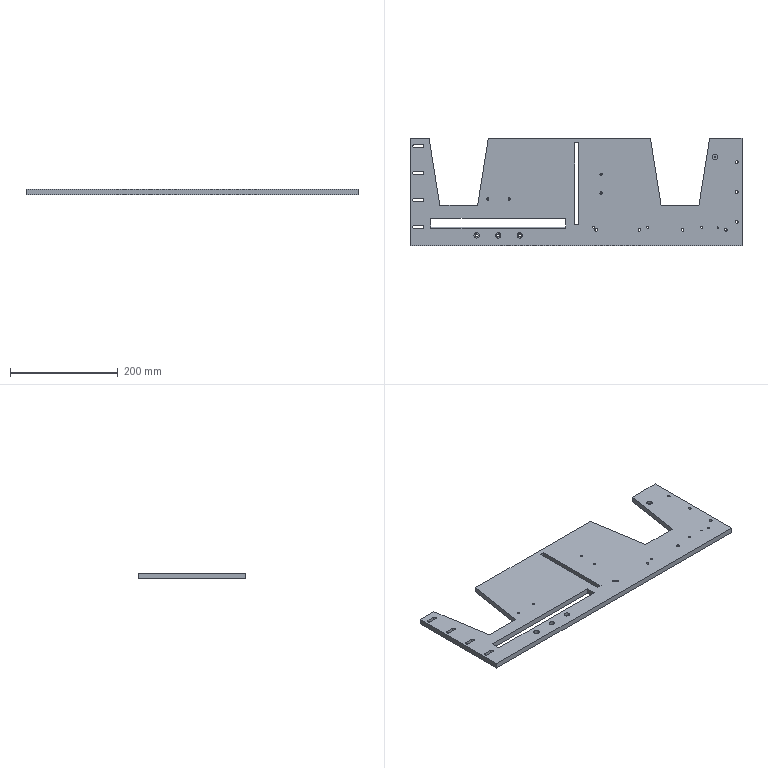Component | SolidWorks | P-SLJ-001-009-2 | 1 solid | 93 faces | box 615 x 200 x 10 mm | volume 943482 mm3 | cylinder 58 | plane 35 | commonest cylinder face diameters 5.5 x24 3.3 x8 10 x8 4.2 x8 5 x8 2.5 x2 | material A3
build123d program:
from build123d import *

# Parameters (mm, degrees)
SKETCH1_W                                            = 615
SKETCH1_H                                            = 200
EXTRUDE1_DEPTH                                       = 5
TAP_DRILL_FOR_M4X0_5_TAP1_D                          = 5.5
EXTRUDE2_DEPTH                                       = 324.506
M6_TAPPED_HOLE1_D                                    = 5
SKETCH9_W                                            = 8
SKETCH9_H                                            = 151
EXTRUDE3_DEPTH                                       = 324.506
EXTRUDE4_DEPTH                                       = 324.506
M5_TAPPED_HOLE1_2_D                                  = 4.2
HOLE_SIZE_ACCORDING_TO_TYPE_OF_HEX_SOCKE_D           = 5.5
HOLE_SIZE_ACCORDING_TO_TYPE_OF_HEX_SOCKE_CBORE_D     = 10
HOLE_SIZE_ACCORDING_TO_TYPE_OF_HEX_SOCKE_CBORE_DEPTH = 5.7
SKETCH16_W                                           = 250
SKETCH16_H                                           = 16
EXTRUDE5_DEPTH                                       = 324.506
M5_TAPPED_HOLE1_D                                    = 4.2
CHAMFER1_SIZE                                        = 2
CHAMFER1_SIZE2                                       = 5
M4_TAPPED_HOLE3_D                                    = 3.3
SKETCH25_R                                           = 5
EXTRUDE6_DEPTH                                       = 5
M4_TAPPED_HOLE4_D                                    = 3.3
M3_TAPPED_HOLE1_D                                    = 2.5


with BuildPart() as part:
    # Sketch1 → Extrude1 (new, symmetric)
    with BuildSketch(Plane.XY):
        Rectangle(SKETCH1_W, SKETCH1_H)
    extrude(amount=EXTRUDE1_DEPTH, both=True)

    # Tap Drill for M4X0.5 Tap1 (through all)
    with Locations(Plane.XY.offset(5)):
        with Locations((297.5, 55), (297.5, 0), (297.5, -55)):
            Hole(TAP_DRILL_FOR_M4X0_5_TAP1_D / 2)

    # Sketch5 → Extrude2 (cut, through all)
    with BuildSketch(Plane.XY.offset(5)):
        Polygon((137.904, 100), (247.5, 100), (227.702, -25), (157.702, -25), align=None)
        Polygon((-272.096, 100), (-162.5, 100), (-182.298, -25), (-252.298, -25), align=None)
    extrude(amount=-EXTRUDE2_DEPTH, mode=Mode.SUBTRACT)

    # M6 Tapped Hole1 (through all)
    with Locations(Plane.XY.offset(5)):
        with Locations((37.5, -70), (117.5, -70), (197.5, -70), (277.5, -70)):
            Hole(M6_TAPPED_HOLE1_D / 2)

    # Sketch9 → Extrude3 (cut, through all)
    with BuildSketch(Plane.XY.offset(5)):
        with Locations((1.5, 15.5)):
            Rectangle(SKETCH9_W, SKETCH9_H)
    extrude(amount=-EXTRUDE3_DEPTH, mode=Mode.SUBTRACT)

    # Sketch10 → Extrude4 (cut, through all)
    with BuildSketch(Plane.XY.offset(5)):
        with BuildLine():
            Line((-300, 87.75), (-285, 87.75))
            ThreePointArc((-285, 87.75), (-282.25, 85), (-285, 82.25))
            Line((-285, 82.25), (-300, 82.25))
            ThreePointArc((-300, 82.25), (-302.75, 85), (-300, 87.75))
        make_face()
        with BuildLine():
            Line((-300, 37.75), (-285, 37.75))
            ThreePointArc((-285, 37.75), (-282.25, 35), (-285, 32.25))
            Line((-285, 32.25), (-300, 32.25))
            ThreePointArc((-300, 32.25), (-302.75, 35), (-300, 37.75))
        make_face()
        with BuildLine():
            Line((-300, -12.25), (-285, -12.25))
            ThreePointArc((-285, -12.25), (-282.25, -15), (-285, -17.75))
            Line((-285, -17.75), (-300, -17.75))
            ThreePointArc((-300, -17.75), (-302.75, -15), (-300, -12.25))
        make_face()
        with BuildLine():
            Line((-300, -62.25), (-285, -62.25))
            ThreePointArc((-285, -62.25), (-282.25, -65), (-285, -67.75))
            Line((-285, -67.75), (-300, -67.75))
            ThreePointArc((-300, -67.75), (-302.75, -65), (-300, -62.25))
        make_face()
    extrude(amount=-EXTRUDE4_DEPTH, mode=Mode.SUBTRACT)

    # M5 Tapped Hole1_2 (through all)
    with Locations(Plane.XY.offset(5)):
        with Locations((-163.5, -13), (-123.5, -13)):
            Hole(M5_TAPPED_HOLE1_2_D / 2)

    # Hole Size_according to_Type of Hex Socke (through all)
    with Locations(Plane(origin=(2.088, 27.304, 5), x_dir=(-1, 0, 0), z_dir=(0, 0, 1))):
        with Locations((186.088, 107.804), (146.088, 107.804), (106.088, 107.804)):
            CounterBoreHole(HOLE_SIZE_ACCORDING_TO_TYPE_OF_HEX_SOCKE_D / 2, HOLE_SIZE_ACCORDING_TO_TYPE_OF_HEX_SOCKE_CBORE_D / 2, HOLE_SIZE_ACCORDING_TO_TYPE_OF_HEX_SOCKE_CBORE_DEPTH)

    # Sketch16 → Extrude5 (cut, through all)
    with BuildSketch(Plane.XY.offset(5)):
        with Locations((-144, -57)):
            Rectangle(SKETCH16_W, SKETCH16_H)
    extrude(amount=-EXTRUDE5_DEPTH, mode=Mode.SUBTRACT)

    # M5 Tapped Hole1 (through all)
    with Locations(Plane.XY.offset(5)):
        with Locations((46.5, 33), (46.5, -2)):
            Hole(M5_TAPPED_HOLE1_D / 2)

    # Chamfer1
    chamfer1_edges = [part.edges().sort_by_distance(p)[0] for p in [
        (-144, -65, 5),
    ]]
    chamfer1_side = [part.faces().sort_by_distance(p)[0] for p in [
        (10.348, -7.574, 5),
    ]]
    chamfer(chamfer1_edges, length=CHAMFER1_SIZE, length2=CHAMFER1_SIZE2, reference=chamfer1_side[0])

    # M4 Tapped Hole3 (through all)
    with Locations(Plane(origin=(0, 0, -5), x_dir=(-1, 0, 0), z_dir=(0, 0, -1))):
        with Locations((-257.5, 65)):
            Hole(M4_TAPPED_HOLE3_D / 2)

    # Sketch25 → Extrude6 (cut)
    with BuildSketch(Plane.XY.offset(5)):
        with Locations((257.5, 65)):
            Circle(SKETCH25_R)
    extrude(amount=-EXTRUDE6_DEPTH, mode=Mode.SUBTRACT)

    # M4 Tapped Hole4 (through all)
    with Locations(Plane.XY.offset(5)):
        with Locations((232.5, -65.5), (132.5, -65.5), (32.5, -65.5)):
            Hole(M4_TAPPED_HOLE4_D / 2)

    # M3 Tapped Hole1 (through all)
    with Locations(Plane.XY.offset(5)):
        with Locations((262.5, -66)):
            Hole(M3_TAPPED_HOLE1_D / 2)


solid = part.part

# Placed as in the assembly
solid = solid.moved(Location((-76, 0, 996.634), (0, 0, 0)))